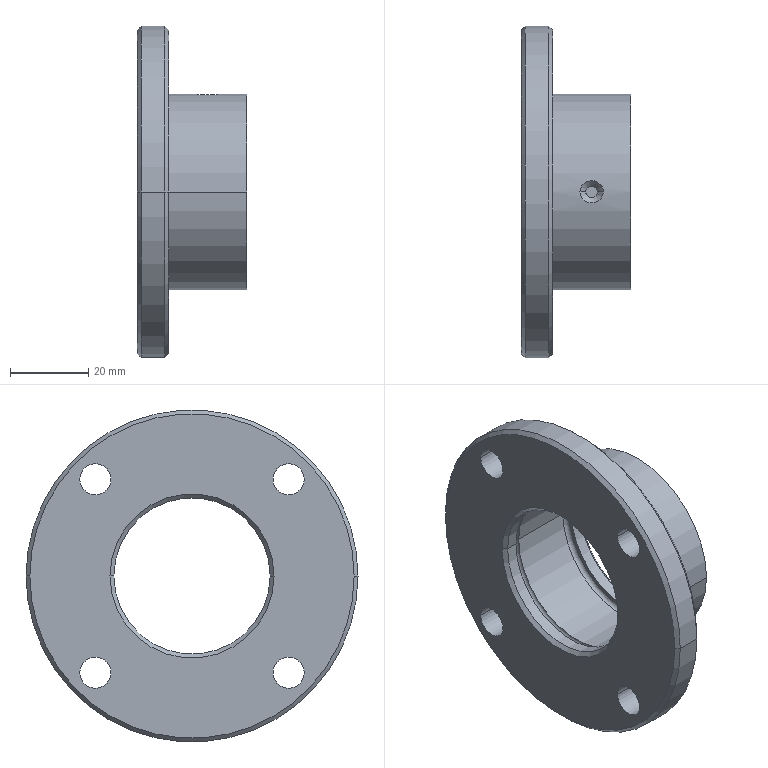Component | SolidWorks | 6Bushing-1 | 1 solid | 39 faces | volume 44439 mm3 | cylinder 20 | cone 10 | plane 5 | torus 4 | commonest cylinder face diameters 8 x8 40 x4 3 x2 42 x2 85 x2 50 x2